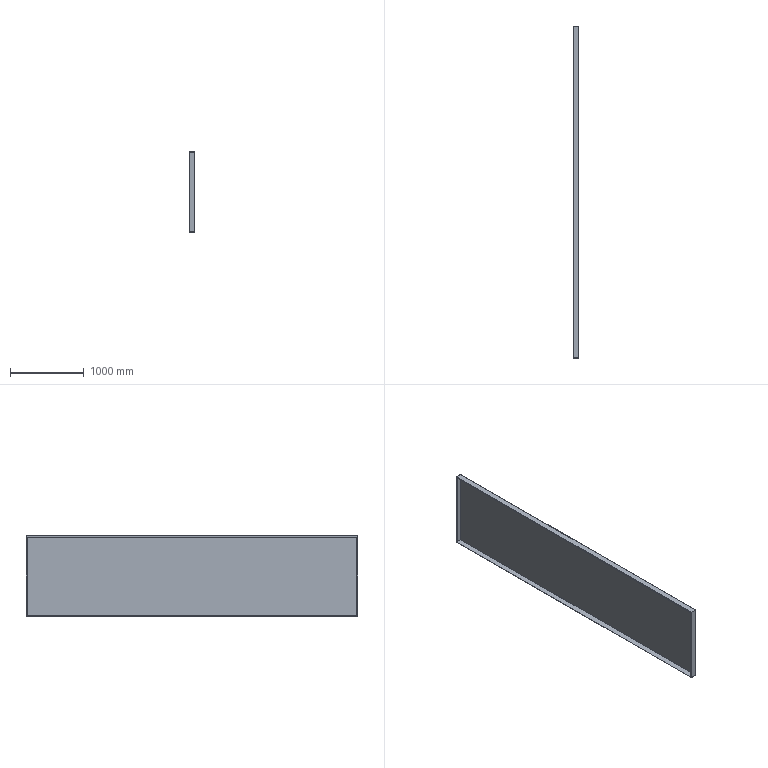Component | NX | CB9 | 1 solid | 15 faces | volume 8772650 mm3 | plane 15